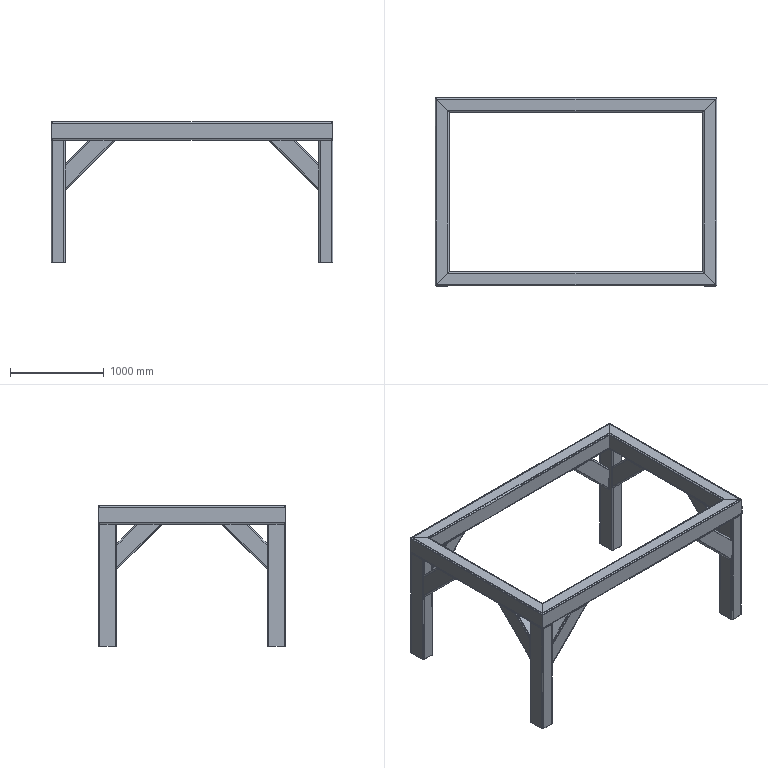Assembly | NX | mm | 16 component files | 16 solids | 288 faces | box 3000 x 2000 x 1500 mm | volume 97086864 mm3 | plane 160 | cylinder 128 | commonest cylinder face diameters 32 x64 16 x64
Bill of materials:
unnamed part 1 | 1 |  | Long straight hollow tube with a rectangular cross-section and rounded corners. Both ends are cut at an angle, giving a trapezoid outline in side view.
unnamed part 2 | 1 |  | Short hollow tube segment with a rectangular cross-section and rounded corners, open at both ends. It is shown tilted relative to the view axes.
unnamed part 3 | 1 |  | Straight hollow tube with a nearly square, rounded-corner rectangular cross-section. It is shown upright and both ends appear cut square.
unnamed part 4 | 1 |  | Long straight hollow tube with a rectangular cross-section and rounded corners. Both ends are cut at an angle, giving a trapezoid side outline that is longer along the top edge.
unnamed part 5 | 1 |  | Long straight hollow tube with a rounded-rectangle cross-section. Both ends are cut at an angle, so one long face is shorter than the opposite face.
unnamed part 6 | 1 |  | Straight hollow tube with a nearly square, rounded-corner rectangular cross-section. It is shown upright and both ends appear cut square.
unnamed part 7 | 1 |  | Short hollow tube segment with a rounded-rectangle cross-section. One open end is visible and the body runs off at an angle, giving a wedge-like outline.
unnamed part 8 | 1 |  | Long straight hollow tube with a rounded-rectangle cross-section. Both ends are cut at an angle, giving a trapezoid outline in one side view.
unnamed part 9 | 1 |  | Short hollow tube segment with a rectangular cross-section and rounded corners, open at both ends. It is shown tilted relative to the view axes.
unnamed part 10 | 1 |  | Short hollow tube segment with a rounded-rectangle cross-section. One open end is visible and the side outlines are slanted.
unnamed part 11 | 1 |  | Short hollow tube segment with a rounded-rectangle cross-section. One open end is visible and the body runs off at an angle, giving a wedge-like outline.
unnamed part 12 | 1 |  | Short hollow tube segment with a rectangular cross-section and rounded corners, open at both ends. It is shown tilted relative to the view axes.
unnamed part 13 | 1 |  | Straight hollow rectangular (near-square) tube with rounded outer and inner corners, uniform thin wall, open at both ends, ends appear cut square to the long axis.
unnamed part 14 | 1 |  | Short hollow rectangular tube with rounded corners and thin uniform wall, with ends that seem to be cut at an angle (mitered) rather than square to the axis.
unnamed part 15 | 1 |  | Hollow rectangular tube with rounded corners and thin uniform wall, open at both ends, with end faces that appear inclined (mitered) relative to the long axis.
unnamed part 16 | 1 |  | Straight hollow rectangular (near-square) tube with rounded outer and inner corners, uniform thin wall, open at both ends, ends appear cut square to the long axis.
Mates:
1. fix | Structure_00_Member_Rectangle_Tube_00 1 component
2. fix | Structure_00_Member_Rectangle_Tube_01 1 component
3. fix | Structure_00_Member_Rectangle_Tube_02 1 component
4. fix | Structure_00_Member_Rectangle_Tube_03 1 component
5. fix | Structure_00_Member_Rectangle_Tube_04 1 component
6. fix | Structure_00_Member_Rectangle_Tube_05 1 component
7. fix | Structure_00_Member_Rectangle_Tube_06 1 component
8. fix | Structure_00_Member_Rectangle_Tube_07 1 component
9. fix | Structure_00_Member_Rectangle_Tube_08 1 component
10. fix | Structure_00_Member_Rectangle_Tube_09 1 component
11. fix | Structure_00_Member_Rectangle_Tube_10 1 component
12. fix | Structure_00_Member_Rectangle_Tube_11 1 component
13. fix | Structure_00_Member_Rectangle_Tube_12 1 component
14. fix | Structure_00_Member_Rectangle_Tube_13 1 component
15. fix | Structure_00_Member_Rectangle_Tube_14 1 component
16. fix | Structure_00_Member_Rectangle_Tube_15 1 component